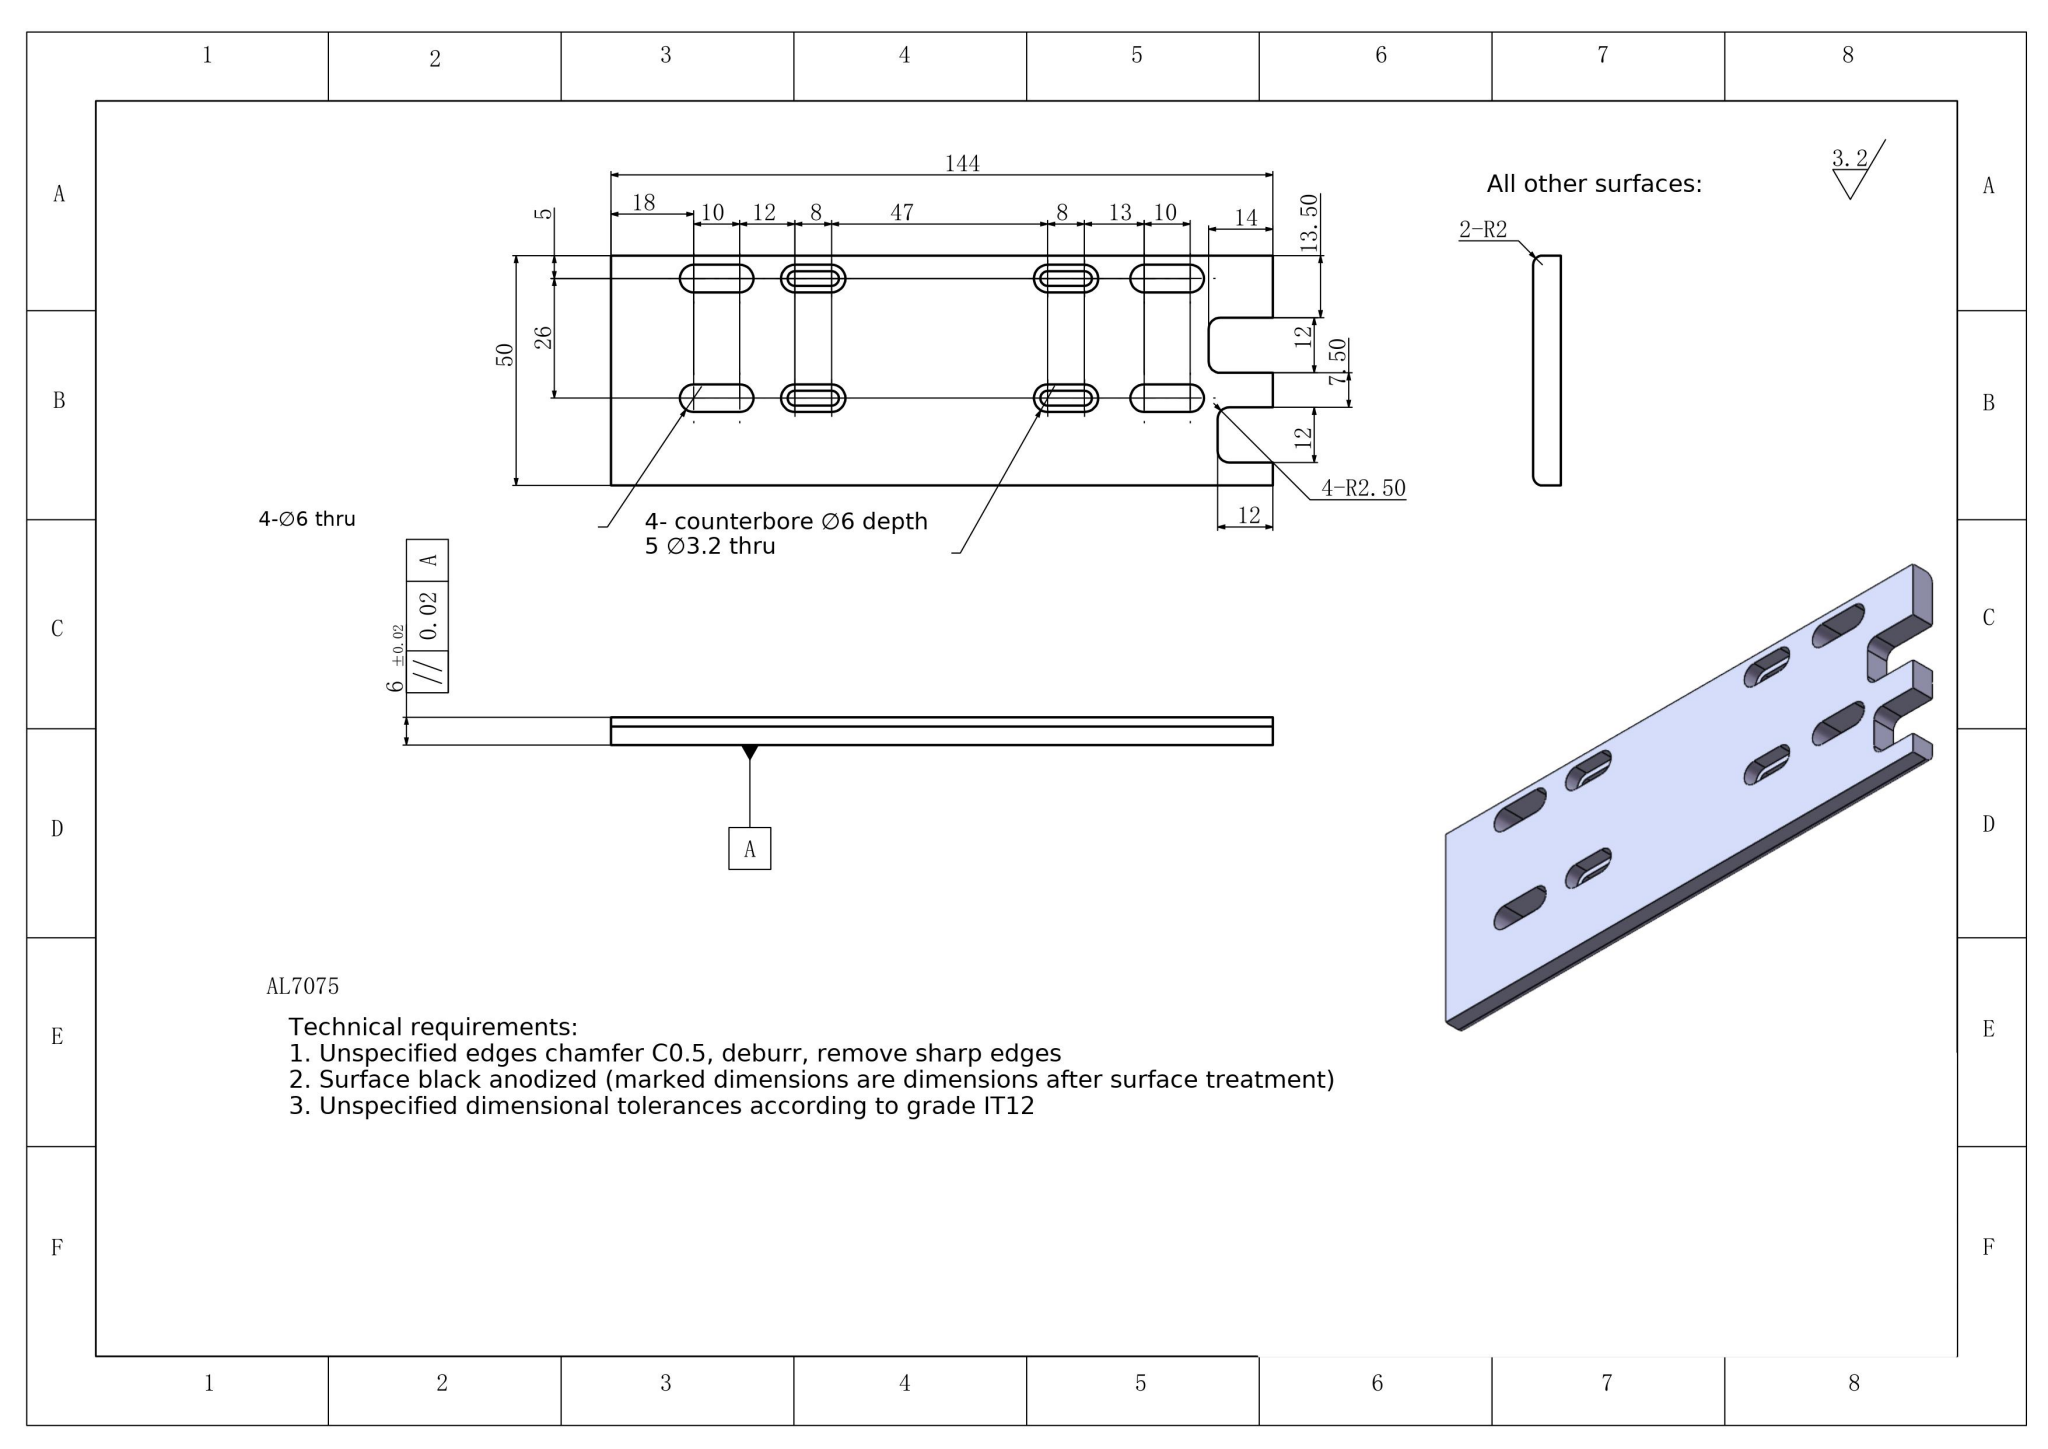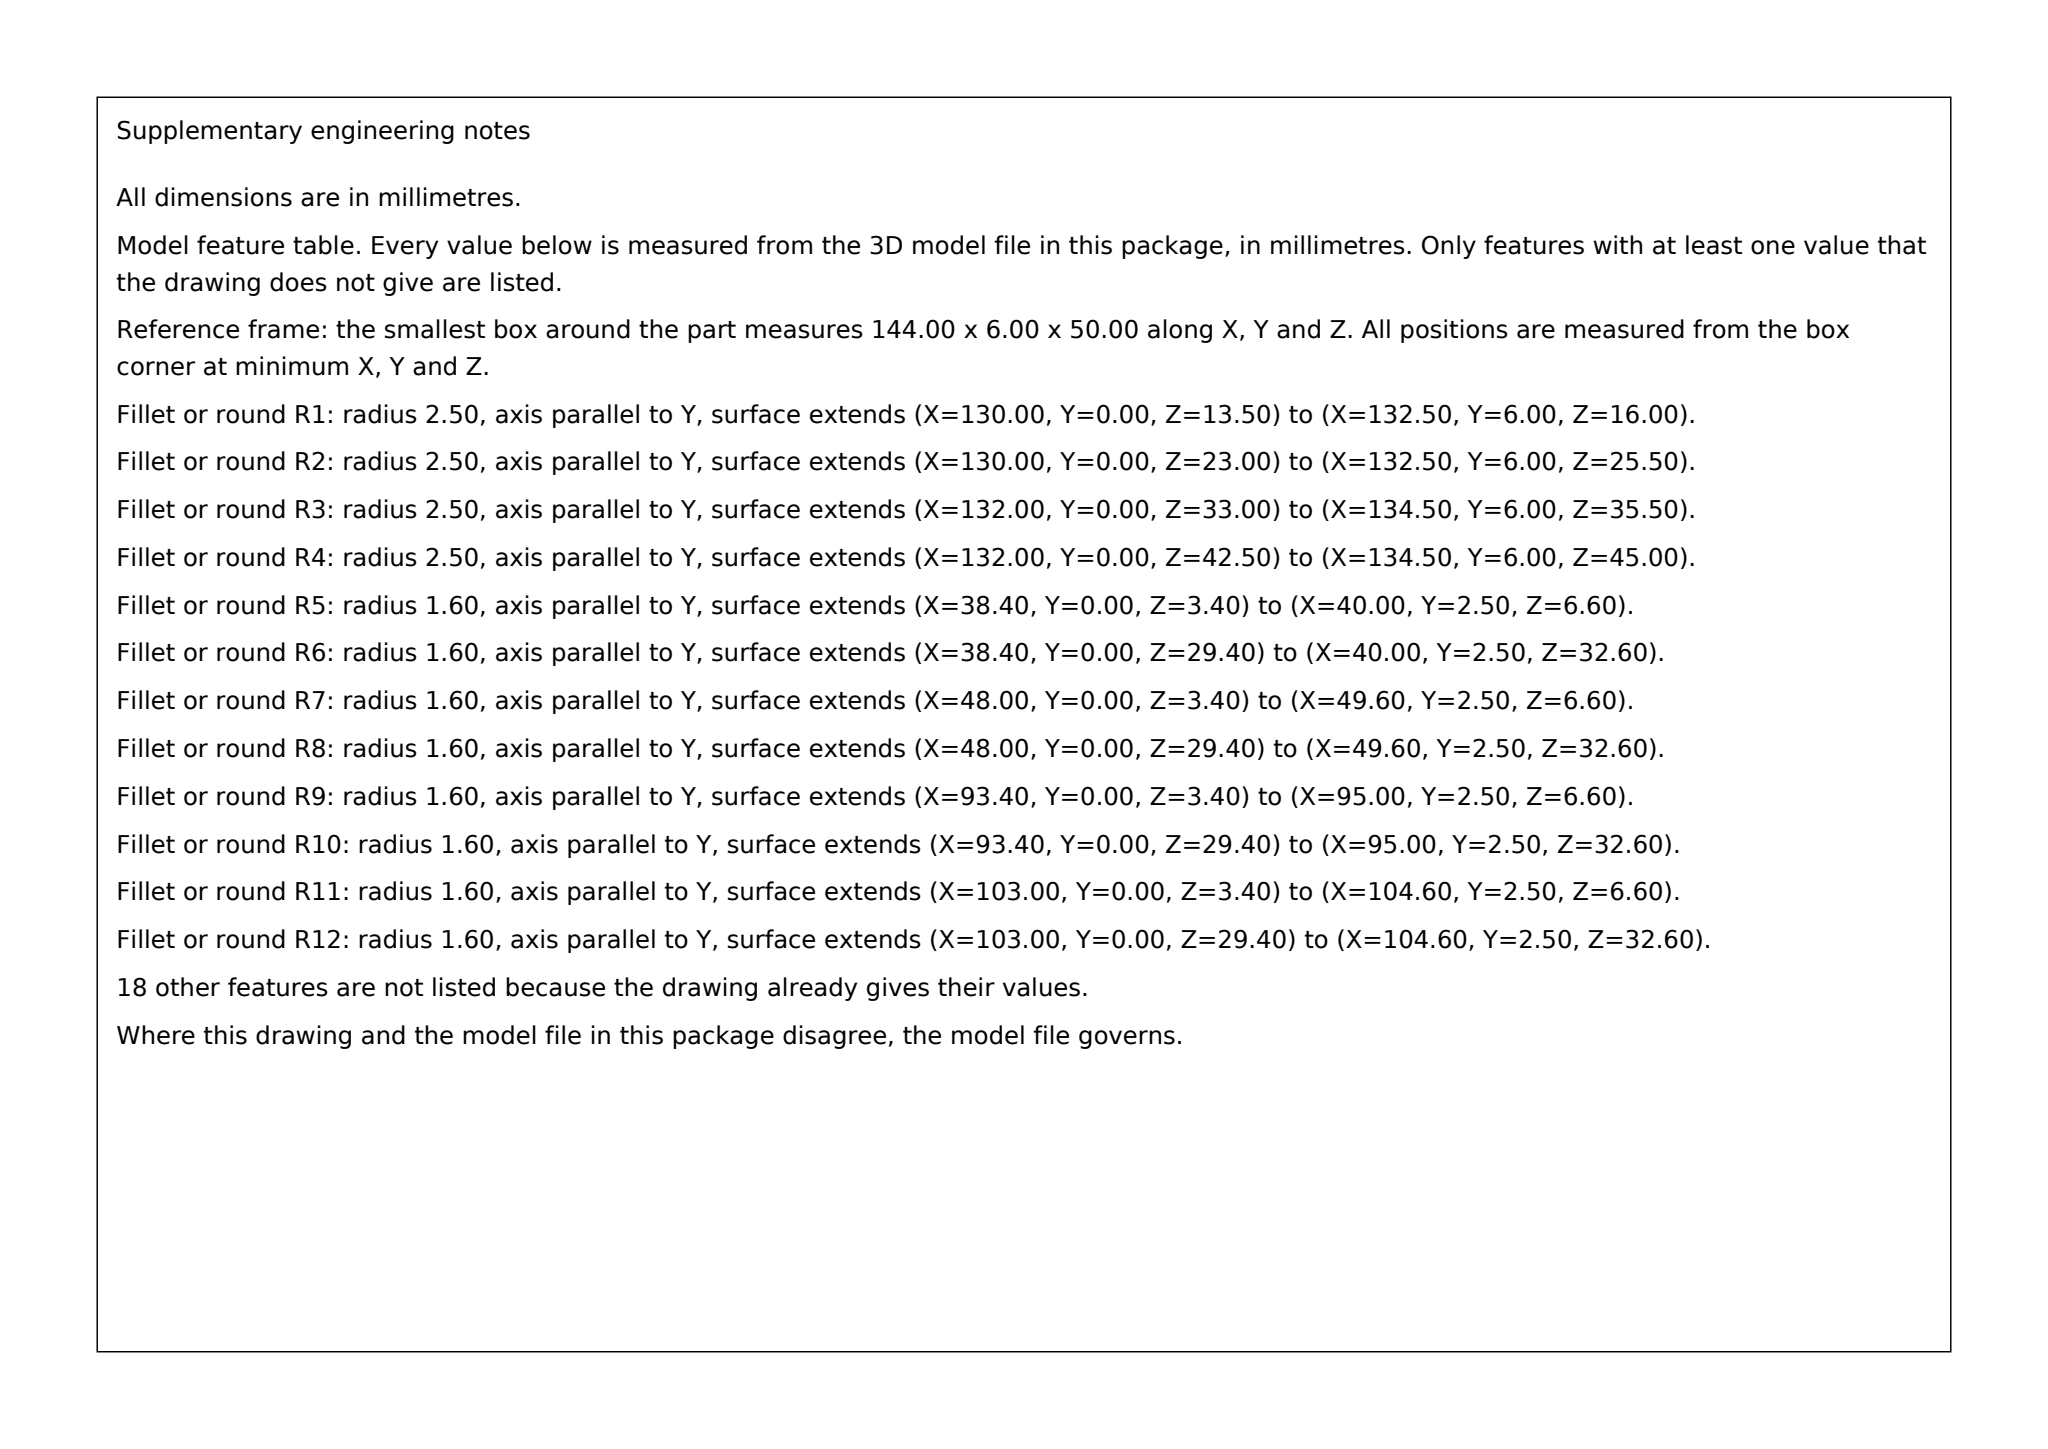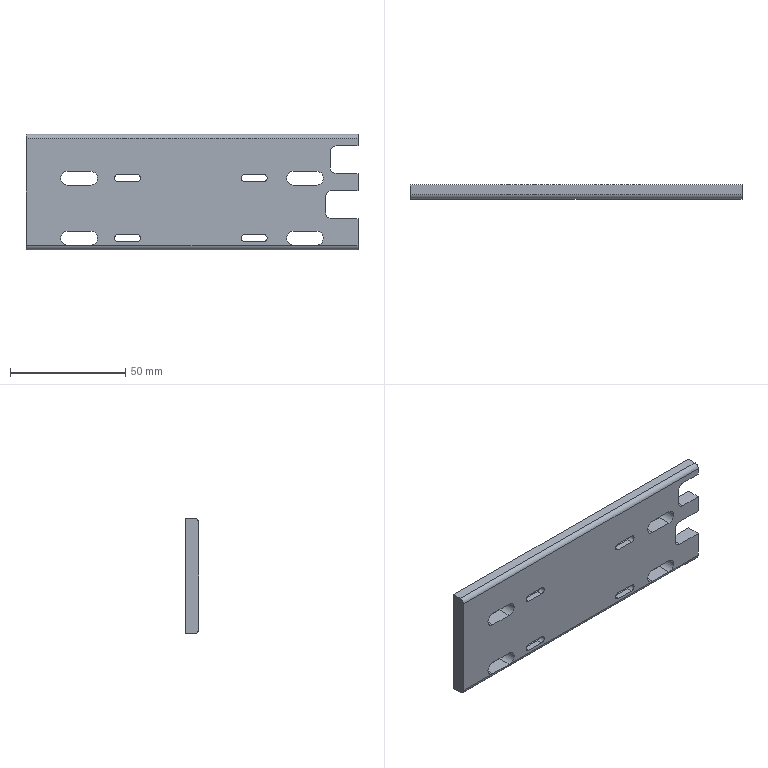Part | SolidWorks | mm | material AL7075 | 1 solid | 76 faces | box 144 x 6 x 50 mm | volume 37590 mm3 | plane 42 | cylinder 34 | commonest cylinder face diameters 6 x20 3.2 x8 5 x4 4 x2
build123d program:
from build123d import *

# Parameters (mm, degrees)
EXTRUDE1_DEPTH          = 50
FILLET1_R               = 2
CUT_EXTRUDE1_DEPTH      = 153.594
CUT_EXTRUDE1_DEPTH_BACK = 153.594
CUT_EXTRUDE2_DEPTH      = 153.67
CUT_EXTRUDE4_DEPTH      = 153.594
CUT_EXTRUDE4_DEPTH_BACK = 153.594
SKETCH7_W               = 20.65
SKETCH7_H               = 12
FILLET2_R               = 2.5
CUT_EXTRUDE5_DEPTH      = 6
CUT_EXTRUDE6_DEPTH      = 153.552
LPATTERN1_COUNT         = 2
LPATTERN1_PITCH         = 98
LPATTERN1_COUNT_DIR2    = 2
LPATTERN1_PITCH_DIR2    = 26
SKETCH10_W              = 241.04
SKETCH10_H              = 148.55
CUT_EXTRUDE7_DEPTH      = 2.5


with BuildPart() as part:
    # Sketch1 → Extrude1 (new body)
    with BuildSketch(Plane.XY):
        Polygon((128.5, 7), (143, 7), (143, 8.5), (144, 8.5), (144, 0), (0, 0), (0, 7), (0, 8.5), (1, 8.5), (1, 7), (15.5, 7), (15.5, 8.5), (16.5, 8.5), (16.5, 7), (31.5, 7), (31.5, 8.5), (32.5, 8.5), (32.5, 7), (47.5, 7), (47.5, 8.5), (48.5, 8.5), (48.5, 7), (63.5, 7), (63.5, 8.5), (64.5, 8.5), (64.5, 7), (79.5, 7), (79.5, 8.5), (80.5, 8.5), (80.5, 7), (95.5, 7), (95.5, 8.5), (96.5, 8.5), (96.5, 7), (111.5, 7), (111.5, 8.5), (112.5, 8.5), (112.5, 7), (127.5, 7), (127.5, 8.5), (128.5, 8.5), align=None)
    extrude(amount=EXTRUDE1_DEPTH)

    # Fillet1
    fillet1_edges = [part.edges().sort_by_distance(p)[0] for p in [
        (72, 0, 50),
        (72, 0, 0),
    ]]
    fillet(fillet1_edges, radius=FILLET1_R)

    # Sketch2 → Cut-Extrude1 (cut, two sides: drawn at the far end of the back side and taken through both)
    with BuildSketch(Plane(origin=(0, 7, 0), x_dir=(1, 0, 0), z_dir=(0, 1, 0)).offset(-CUT_EXTRUDE1_DEPTH_BACK)):
        with BuildLine():
            Line((158.814, -13.5), (132.5, -13.5))
            ThreePointArc((132.5, -13.5), (130.732, -14.232), (130, -16))
            Line((130, -16), (130, -23))
            ThreePointArc((130, -23), (130.732, -24.768), (132.5, -25.5))
            Line((132.5, -25.5), (158.814, -25.5))
            Line((158.814, -25.5), (158.814, -13.5))
        make_face()
    extrude(amount=CUT_EXTRUDE1_DEPTH + CUT_EXTRUDE1_DEPTH_BACK, mode=Mode.SUBTRACT)

    # Sketch5 → Cut-Extrude2 (cut, through all)
    with BuildSketch(Plane(origin=(0, 8.5, 0), x_dir=(1, 0, 0), z_dir=(0, 1, 0))):
        with BuildLine():
            Line((18, -2), (28, -2))
            ThreePointArc((28, -2), (31, -5), (28, -8))
            Line((28, -8), (18, -8))
            ThreePointArc((18, -8), (15, -5), (18, -2))
        make_face()
    cut_extrude2 = extrude(amount=-CUT_EXTRUDE2_DEPTH, mode=Mode.SUBTRACT)

    # Sketch7 → Cut-Extrude4 (cut, two sides: drawn at the far end of the back side and taken through both)
    with BuildSketch(Plane(origin=(0, 7, 0), x_dir=(1, 0, 0), z_dir=(0, 1, 0)).offset(-CUT_EXTRUDE4_DEPTH_BACK)):
        with Locations((142.325, -39)):
            Rectangle(SKETCH7_W, SKETCH7_H)
    extrude(amount=CUT_EXTRUDE4_DEPTH + CUT_EXTRUDE4_DEPTH_BACK, mode=Mode.SUBTRACT)

    # Fillet2
    fillet2_edges = [part.edges().sort_by_distance(p)[0] for p in [
        (132, 3.5, 45),
        (132, 3.5, 33),
    ]]
    fillet(fillet2_edges, radius=FILLET2_R)

    # Sketch8 → Cut-Extrude5 (cut)
    with BuildSketch(Plane(origin=(0, 8.5, 0), x_dir=(1, 0, 0), z_dir=(0, 1, 0))):
        with BuildLine():
            Line((40, -2), (48, -2))
            ThreePointArc((48, -2), (51, -5), (48, -8))
            Line((48, -8), (40, -8))
            ThreePointArc((40, -8), (37, -5), (40, -2))
        make_face()
        with BuildLine():
            Line((40, -28), (48, -28))
            ThreePointArc((48, -28), (51, -31), (48, -34))
            Line((48, -34), (40, -34))
            ThreePointArc((40, -34), (37, -31), (40, -28))
        make_face()
        with BuildLine():
            Line((95, -2), (103, -2))
            ThreePointArc((103, -2), (106, -5), (103, -8))
            Line((103, -8), (95, -8))
            ThreePointArc((95, -8), (92, -5), (95, -2))
        make_face()
        with BuildLine():
            Line((95, -28), (103, -28))
            ThreePointArc((103, -28), (106, -31), (103, -34))
            Line((103, -34), (95, -34))
            ThreePointArc((95, -34), (92, -31), (95, -28))
        make_face()
    extrude(amount=-CUT_EXTRUDE5_DEPTH, mode=Mode.SUBTRACT)

    # Sketch9 → Cut-Extrude6 (cut, through all)
    with BuildSketch(Plane(origin=(0, 2.5, 0), x_dir=(1, 0, 0), z_dir=(0, 1, 0))):
        with BuildLine():
            Line((48, -3.4), (40, -3.4))
            ThreePointArc((40, -3.4), (38.4, -5), (40, -6.6))
            Line((40, -6.6), (48, -6.6))
            ThreePointArc((48, -6.6), (49.6, -5), (48, -3.4))
        make_face()
        with BuildLine():
            Line((95, -6.6), (103, -6.6))
            ThreePointArc((103, -6.6), (104.6, -5), (103, -3.4))
            Line((103, -3.4), (95, -3.4))
            ThreePointArc((95, -3.4), (93.4, -5), (95, -6.6))
        make_face()
        with BuildLine():
            Line((40, -32.6), (48, -32.6))
            ThreePointArc((48, -32.6), (49.6, -31), (48, -29.4))
            Line((48, -29.4), (40, -29.4))
            ThreePointArc((40, -29.4), (38.4, -31), (40, -32.6))
        make_face()
        with BuildLine():
            Line((95, -32.6), (103, -32.6))
            ThreePointArc((103, -32.6), (104.6, -31), (103, -29.4))
            Line((103, -29.4), (95, -29.4))
            ThreePointArc((95, -29.4), (93.4, -31), (95, -32.6))
        make_face()
    extrude(amount=-CUT_EXTRUDE6_DEPTH, mode=Mode.SUBTRACT)

    # LPattern1: Cut-Extrude2 2 × 2
    with Locations(*[(i * LPATTERN1_PITCH, 0, j * LPATTERN1_PITCH_DIR2) for i in range(LPATTERN1_COUNT) for j in range(LPATTERN1_COUNT_DIR2) if (i, j) != (0, 0)]):
        add(cut_extrude2, mode=Mode.SUBTRACT)

    # Sketch10 → Cut-Extrude7 (cut)
    with BuildSketch(Plane(origin=(0, 8.5, 0), x_dir=(1, 0, 0), z_dir=(0, 1, 0))):
        with Locations((80.088, -28.684)):
            Rectangle(SKETCH10_W, SKETCH10_H)
    extrude(amount=-CUT_EXTRUDE7_DEPTH, mode=Mode.SUBTRACT)


solid = part.part